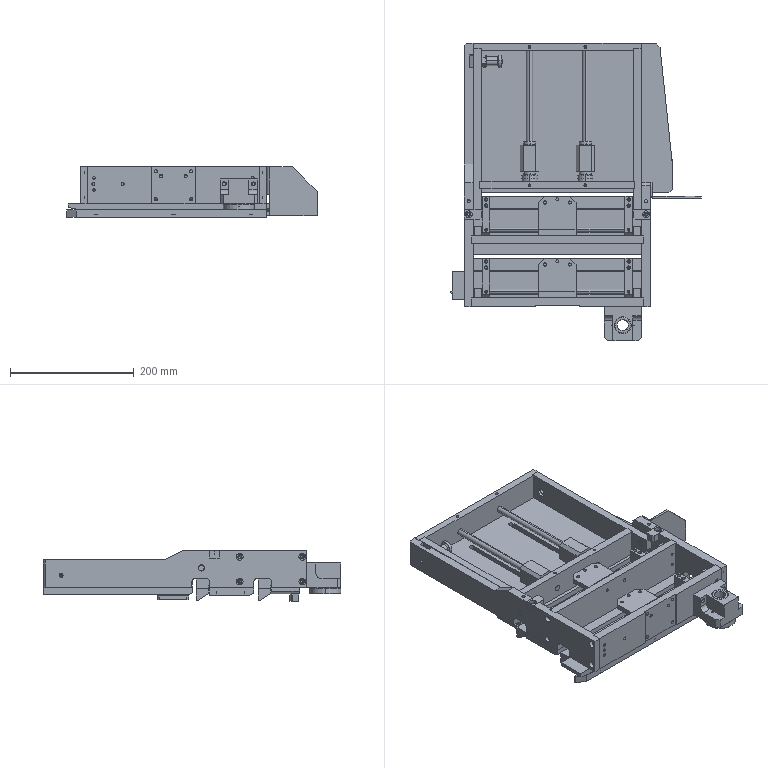Assembly | SolidWorks | mm | 48 component files | 48 solids | 1236 faces | box 404 x 480 x 82 mm | volume 3316165 mm3 | cylinder 579 | plane 451 | cone 200 | torus 4 | sphere 2 | commonest cylinder face diameters 5 x80 4.2 x78 10 x76 5.5 x62 6.6 x44 11 x42 12 x38 8 x28
Bill of materials:
LML10UU | 2 |  | Hollow cylindrical tube/sleeve with a through bore, chamfered ends and two shallow circumferential grooves near each end.
OPW-05-001 | 1 |  | Thick flat plate with an irregular stepped outline: a rectangular notch in one long edge, rounded-corner cutouts in the opposite edge, a chamfered corner, and several through holes including one larger hole near one end.
OPW-05-002 | 1 |  | Long thick bar/plate with a stepped and sloped top profile, rectangular notch, two rounded cutouts on the lower edge, multiple small through holes, one larger hole, and a rectangular pocket/recess near one end.
OPW-05-003 | 1 |  | Long rectangular bar with a shallow step/recess on one face in the middle section and a pattern of small holes on the main face plus two larger holes on each end face.
OPW-05-005 | 1 |  | Plain long rectangular bar with six small holes on the main face and two blind holes in each end face.
OPW-05-006 | 1 |  | Thin flat rectangular plate with one angled/chamfered corner, six small through holes and two larger holes that appear counterbored or larger near the ends.
OPW-05-007 | 1 |  | Thin flat plate of roughly rectangular outline with one long tapered/angled edge and chamfered corners, two long parallel slots, and six small holes along two opposite edges.
OPW-05-008 | 1 |  | Thin flat rectangular frame-like plate with three rounded-rectangular through windows separated by narrow webs, each web having two small holes, and chamfered outer corners.
OPW-05-010 | 1 |  | Prismatic block with a large vertical through bore, a raised central section with a curved (radiused) inner transition, stepped side ledges, horizontal cross holes, and chamfered corners on one end.
OPW-05-011 | 1 | Brass | Flanged cylindrical bushing: a hollow cylindrical body with a coaxial bore and a round flange at one end with four equally spaced through holes.
OPW-05-014 | 1 |  | Long slender rectangular bar with one angled/pointed end and three evenly spaced small holes along its length.
OPW-05-033 | 1 |  | Bent sheet-metal bracket with an L-shaped cross-section: a larger plate with an angled corner and a short perpendicular flange containing two holes.
STB-08-024 | 1 |  | Axisymmetric part with a hexagonal body at one end and a stepped cylindrical shank; a bore runs through along the axis.
STB-08-025 | 1 |  | Long cylindrical pin with a single raised annular collar near one end.
STB-08-026 | 1 |  | Short hollow cylindrical ring or sleeve with a central through bore.
STB-08-027 | 1 |  | Headed pin: a plain cylindrical shank with a larger-diameter head that has a domed outer face.
STB-08-005 | 1 |  | Long, thin, flat rectangular bar with a group of holes at each end and small holes along its length.
STB-08-007 | 2 | Brass | Long, slender prismatic bar with a non-rectangular cross-section (one sloped side ending in a rounded tip) and several holes.
STB-08-008 | 4 |  | Rectangular block with two parallel holes in one face and one larger perpendicular hole in an adjacent face.
STB-08-009 | 4 |  | Elongated rectangular block with one end chamfered, a transverse through hole at that end, top holes, and a stepped underside.
STB-08-010 | 2 |  | Long, slender, plain cylindrical rod.
STB-08-011 | 2 |  | Block with an L-shaped side profile: a thicker upright section at one end and a thinner base, with chamfered plan corners and several holes.
STB-08-015 | 2 |  | Solid plain cylinder with chamfered edges at both ends.
STB-08-020 | 2 |  | Long, slender, plain cylindrical rod, similar in form to a thin pin or wire segment.
STB-08-021 | 2 |  | Prismatic block with a large cylindrical through-bore along its length; the cross-section is a rectangle with two chamfered top corners, and a narrower rectangular tab hangs below it. The tab runs only part of the block's length, so the side profile is L-shaped.
STB-08-022 | 4 |  | Flat annular ring (washer-like disc) with a concentric central through-hole and plain cylindrical outer and inner surfaces.
STB-08-042 | 1 | 6061 Alloy | Long, thin rectangular bar. One end has a stepped L-shaped notch with a small chamfer and an inside fillet. There is one larger through-hole near each end and two smaller through-holes next to the notched end. A small raised or stepped tab detail sits near the notched end on one side face.
STB-08-042JX | 1 | 6061 Alloy | Long, thin rectangular bar with an L-shaped notch at one end (small chamfer and inside fillet). It has a larger through-hole near each end and two smaller through-holes beside the notched end. A small step appears on the face opposite the one seen on the similar part.
STB-08-043 | 1 | 6061 Alloy | Long rectangular bar with two through-holes in the main face, spaced along its length. It also has two small holes in the top narrow edge and two small holes in one end face.
STB-08-044 | 1 |  | Long rectangular bar with stepped (rebated) ends: a narrower raised strip runs along one long face between the end steps. It has two through-holes in the main face, two small holes near each end of the face, two small holes in the top edge, and small holes in both end faces.
STB-08-045 | 2 |  | Rectangular block with two chamfered corners at one end in plan view and a counterbored vertical through-hole near the other end.
Mates:
1. concentric | OPW-05-003-1 face at (-243.904, 48.999, -20) dir (-1, 0, 0) r 2.5 | OPW-05-002-1 face at (-254.904, 48.999, -20) dir (-1, 0, 0) r 3.3
2. concentric | OPW-05-003-1 face at (-243.904, 48.999, 20) dir (-1, 0, 0) r 2.5 | OPW-05-002-1 face at (-254.904, 48.999, 20) dir (-1, 0, 0) r 3.3
3. coincident | OPW-05-003-1 face at (-243.904, 55.999, -30) dir (-1, 0, 0) | OPW-05-002-1 face at (-243.904, 55.999, -30) dir (1, 0, 0)
4. concentric | OPW-05-003-1 face at (34.096, 48.999, -20) dir (1, 0, 0) r 2.5 | OPW-05-001-1 face at (45.096, 48.999, -20) dir (1, 0, 0) r 5.5
5. concentric | OPW-05-003-1 face at (34.096, 48.999, 20) dir (1, 0, 0) r 2.5 | OPW-05-001-1 face at (45.096, 48.999, 20) dir (1, 0, 0) r 5.5
6. coincident | OPW-05-003-1 face at (34.096, 55.999, -30) dir (1, 0, 0) | OPW-05-001-1 face at (34.096, 55.999, -30) dir (-1, 0, 0)
7. concentric | OPW-05-002-1 face at (-254.904, 149.999, 20) dir (-1, 0, 0) r 5.5 | OPW-05-005-1 face at (-243.904, 149.999, 20) dir (-1, 0, 0) r 2.5
8. concentric | OPW-05-002-1 face at (-254.904, 149.999, -20) dir (-1, 0, 0) r 5.5 | OPW-05-005-1 face at (-243.904, 149.999, -20) dir (-1, 0, 0) r 2.5
9. coincident | OPW-05-002-1 face at (-243.904, 143.999, 30) dir (1, 0, 0) | OPW-05-005-1 face at (-243.904, 155.999, -30) dir (-1, 0, 0)
10. concentric | OPW-05-003-1 face at (-232.904, 55.999, -8) dir (0, 1, 0) r 2.1 | STB-08-008-1 face at (-232.904, 71.999, -8) dir (0, 1, 0) r 2.75
11. concentric | OPW-05-003-1 face at (-232.904, 55.999, 12) dir (0, 1, 0) r 2.1 | STB-08-008-1 face at (-232.904, 71.999, 12) dir (0, 1, 0) r 2.75
12. coincident | OPW-05-003-1 face at (-243.904, 55.999, 30) dir (0, 1, 0) | STB-08-008-1 face at (-238.904, 55.999, -27) dir (0, -1, 0)
13. concentric | OPW-05-003-1 face at (23.096, 55.999, 12) dir (0, 1, 0) r 2.1 | STB-08-008-2 face at (23.096, 71.999, 12) dir (0, 1, 0) r 2.75
14. concentric | OPW-05-003-1 face at (23.096, 55.999, -8) dir (0, 1, 0) r 2.1 | STB-08-008-2 face at (23.096, 71.999, -8) dir (0, 1, 0) r 2.75
15. coincident | OPW-05-003-1 face at (-243.904, 55.999, 30) dir (0, 1, 0) | STB-08-008-2 face at (17.096, 55.999, -27) dir (0, -1, 0)
16. concentric | OPW-05-005-1 face at (23.096, 155.999, 12) dir (0, 1, 0) r 2.1 | STB-08-008-4 face at (23.096, 171.999, 12) dir (0, 1, 0) r 2.75
17. concentric | OPW-05-005-1 face at (23.096, 155.999, -8) dir (0, 1, 0) r 2.1 | STB-08-008-4 face at (23.096, 171.999, -8) dir (0, 1, 0) r 2.75
18. coincident | OPW-05-005-1 face at (-243.904, 155.999, 30) dir (0, 1, 0) | STB-08-008-4 face at (17.096, 155.999, -27) dir (0, -1, 0)
19. concentric | OPW-05-005-1 face at (-232.904, 155.999, -8) dir (0, 1, 0) r 2.1 | STB-08-008-3 face at (-232.904, 171.999, -8) dir (0, 1, 0) r 2.75
20. concentric | OPW-05-005-1 face at (-232.904, 155.999, 12) dir (0, 1, 0) r 2.1 | STB-08-008-3 face at (-232.904, 171.999, 12) dir (0, 1, 0) r 2.75
21. coincident | OPW-05-005-1 face at (-243.904, 155.999, 30) dir (0, 1, 0) | STB-08-008-3 face at (-238.904, 155.999, -27) dir (0, -1, 0)
22. concentric | STB-08-010-1 face at (29.096, 65.999, -19) dir (-1, 0, 0) r 4 | STB-08-008-2 face at (17.095, 65.999, -19) dir (1, 0, 0) r 4
23. coincident | STB-08-010-1 face at (29.096, 65.999, -19) dir (1, 0, 0) | STB-08-008-2 face at (29.096, 55.999, -27) dir (1, 0, 0)
24. concentric | STB-08-009-1 face at (-225.905, 65.999, -19) dir (1, 0, 0) r 4 | STB-08-010-1 face at (29.096, 65.999, -19) dir (-1, 0, 0) r 4
25. concentric | STB-08-007-1 face at (-219.904, 114.999, -31) dir (0, 0, 1) r 2.1 | STB-08-009-1 face at (-219.904, 114.999, -9) dir (0, 0, 1) r 2.75
26. concentric | STB-08-007-1 face at (-219.904, 104.999, -31) dir (0, 0, 1) r 2.1 | STB-08-009-1 face at (-219.904, 104.999, -9) dir (0, 0, 1) r 2.75
27. coincident | STB-08-007-1 face at (-254.904, 119.999, -31) dir (0, 0, 1) | STB-08-009-1 face at (-225.904, 57.999, -31) dir (0, 0, -1)
28. concentric | STB-08-007-1 face at (10.096, 104.999, -31) dir (0, 0, 1) r 2.1 | STB-08-009-2 face at (10.096, 104.999, -9) dir (0, 0, 1) r 2.75
29. concentric | STB-08-007-1 face at (10.096, 114.999, -31) dir (0, 0, 1) r 2.1 | STB-08-009-2 face at (10.096, 114.999, -9) dir (0, 0, 1) r 2.75
30. coincident | STB-08-007-1 face at (-254.904, 119.999, -31) dir (0, 0, 1) | STB-08-009-2 edge at (10.096, 104.999, -31) dir (0, 0, 1) r 2.75
31. distance | STB-08-008-1 face at (-226.904, 55.999, -27) dir (1, 0, 0) | STB-08-009-1 face at (-225.904, 119.999, -9) dir (-1, 0, 0)
32. parallel | OPW-05-002-1 face at (-240.903, 98.999, -30) dir (0, 1, 0) | STB-08-007-1 face at (-254.904, 119.999, -51) dir (0, 1, 0)
33. concentric | OPW-05-003-1 face at (-124.904, 55.999, 15) dir (0, 1, 0) r 2.5 | STB-08-011-1 face at (-124.904, 65.999, 15) dir (0, 1, 0) r 3.5
34. concentric | OPW-05-003-1 face at (-84.904, 55.999, 15) dir (0, 1, 0) r 2.5 | STB-08-011-1 face at (-84.904, 65.999, 15) dir (0, 1, 0) r 3.5
35. coincident | OPW-05-003-1 face at (-243.904, 55.999, 30) dir (0, 1, 0) | STB-08-011-1 face at (-134.904, 55.999, 1) dir (0, -1, 0)
36. concentric | STB-08-008-3 face at (-238.905, 165.999, -19) dir (1, 0, 0) r 4 | STB-08-010-2 face at (29.096, 165.999, -19) dir (-1, 0, 0) r 4
37. coincident | STB-08-008-3 face at (-238.904, 155.999, -27) dir (-1, 0, 0) | STB-08-010-2 face at (-238.904, 165.999, -19) dir (-1, 0, 0)
38. concentric | STB-08-009-3 face at (-225.905, 165.999, -19) dir (1, 0, 0) r 4 | STB-08-010-2 face at (29.096, 165.999, -19) dir (-1, 0, 0) r 4
39. concentric | STB-08-007-2 face at (-219.904, 214.999, -31) dir (0, 0, 1) r 2.1 | STB-08-009-3 face at (-219.904, 214.999, -9) dir (0, 0, 1) r 2.75
40. concentric | STB-08-007-2 face at (10.096, 214.999, -31) dir (0, 0, 1) r 2.1 | STB-08-009-4 face at (10.096, 214.999, -9) dir (0, 0, 1) r 2.75
41. coincident | STB-08-009-4 edge at (4.096, 165.999, -19) dir (-1, 0, 0) r 4 | STB-08-010-2 face at (29.096, 165.999, -19) dir (-1, 0, 0) r 4
42. coincident | STB-08-007-2 face at (-254.904, 219.999, -31) dir (0, 0, 1) | STB-08-009-4 edge at (10.096, 204.999, -31) dir (0, 0, 1) r 2.75
43. parallel | OPW-05-002-1 face at (-240.903, 198.999, -30) dir (0, 1, 0) | STB-08-007-2 face at (-254.904, 219.999, -51) dir (0, 1, 0)
44. coincident | STB-08-007-1 face at (-254.904, 99.999, -51) dir (-1, 0, 0) | STB-08-007-2 face at (-254.904, 199.999, -51) dir (-1, 0, 0)
45. concentric | OPW-05-005-1 face at (-84.904, 155.999, 15) dir (0, 1, 0) r 2.5 | STB-08-011-2 face at (-84.904, 165.999, 15) dir (0, 1, 0) r 3.5
46. concentric | OPW-05-005-1 face at (-124.904, 155.999, 15) dir (0, 1, 0) r 2.5 | STB-08-011-2 face at (-124.904, 165.999, 15) dir (0, 1, 0) r 3.5
47. coincident | OPW-05-005-1 face at (-243.904, 155.999, 30) dir (0, 1, 0) | STB-08-011-2 face at (-134.904, 155.999, 1) dir (0, -1, 0)
48. concentric | OPW-05-001-1 face at (38.096, 90.999, -30) dir (0, 0, -1) r 2.5 | STB-08-005-1 face at (38.096, 90.999, -40) dir (0, 0, -1) r 5.5
49. concentric | OPW-05-001-1 face at (38.096, 72.999, -30) dir (0, 0, -1) r 2.5 | STB-08-005-1 face at (38.096, 72.999, -40) dir (0, 0, -1) r 5.5
50. coincident | OPW-05-001-1 face at (31.096, 241.999, -30) dir (0, 0, -1) | STB-08-005-1 face at (45.096, 53.999, -30) dir (0, 0, 1)
51. concentric | STB-08-005-1 face at (20.096, 60.999, -40) dir (0, 0, -1) r 2.1 | OPW-05-014-1 face at (20.096, 60.999, -52) dir (0, 0, -1) r 2.75
52. concentric | STB-08-005-1 face at (-104.904, 60.999, -40) dir (0, 0, -1) r 2.1 | OPW-05-014-1 face at (-104.904, 60.999, -52) dir (0, 0, -1) r 2.75
53. coincident | STB-08-005-1 face at (45.096, 53.999, -40) dir (0, 0, -1) | OPW-05-014-1 face at (45.096, 54.999, -40) dir (0, 0, 1)
54. concentric | OPW-05-002-1 face at (-247.904, 190.999, 18) dir (0, 0, 1) r 2.5 | STB-08-045-1 face at (-247.904, 190.999, 30) dir (0, 0, 1) r 3.3
55. coincident | OPW-05-002-1 face at (-254.904, 198.999, 18) dir (0, 0, 1) | STB-08-045-1 face at (-254.904, 182.999, 18) dir (0, 0, -1)
56. coincident | OPW-05-002-1 face at (-254.904, 41.999, -30) dir (-1, 0, 0) | STB-08-045-1 face at (-254.904, 198.999, 30) dir (-1, 0, 0)
57. concentric | OPW-05-001-1 face at (38.096, 190.999, 18) dir (0, 0, 1) r 2.5 | STB-08-045-2 face at (38.096, 190.999, 30) dir (0, 0, 1) r 3.3
58. coincident | OPW-05-001-1 face at (31.095, 198.999, 18) dir (0, 0, 1) | STB-08-045-2 face at (45.096, 198.999, 18) dir (0, 0, -1)
59. coincident | OPW-05-001-1 face at (45.096, 41.999, -30) dir (1, 0, 0) | STB-08-045-2 face at (45.096, 182.999, 30) dir (1, 0, 0)
60. concentric | OPW-05-002-1 face at (-247.904, 186.999, -30) dir (0, 0, -1) r 2.5 | OPW-05-006-1 face at (-247.904, 186.999, -42) dir (0, 0, -1) r 3.3
61. concentric | OPW-05-002-1 face at (-247.904, 141.999, -30) dir (0, 0, -1) r 2.5 | OPW-05-006-1 face at (-247.904, 141.999, -42) dir (0, 0, -1) r 3.3
62. coincident | OPW-05-002-1 face at (-254.904, 466.999, -30) dir (0, 0, -1) | OPW-05-006-1 face at (45.096, 126.999, -30) dir (0, 0, 1)
63. concentric | OPW-05-002-1 face at (-254.905, 211.999, 2) dir (1, 0, 0) r 5 | STB-08-042-1 face at (-227.903, 211.999, 2) dir (-1, 0, 0) r 6
64. concentric | OPW-05-001-1 face at (31.095, 211.999, 2) dir (1, 0, 0) r 5 | STB-08-042JX-1 face at (18.095, 211.999, 2) dir (1, 0, 0) r 6
65. concentric | STB-08-042-1 face at (-233.904, 457.999, 5.5) dir (0, 1, 0) r 2.1 | STB-08-044-1 face at (-233.904, 466.999, 5.5) dir (0, 1, 0) r 5
66. concentric | STB-08-042-1 face at (-233.904, 457.999, -19.5) dir (0, 1, 0) r 2.1 | STB-08-044-1 face at (-233.904, 466.999, -19.5) dir (0, 1, 0) r 2.75
67. coincident | STB-08-042-1 face at (-239.904, 457.999, -29) dir (0, 1, 0) | STB-08-044-1 face at (-239.904, 457.999, -29.001) dir (0, -1, 0)
68. concentric | STB-08-042JX-1 face at (24.096, 457.999, -19.5) dir (0, 1, 0) r 2.1 | STB-08-044-1 face at (24.096, 466.999, -19.5) dir (0, 1, 0) r 5
69. concentric | STB-08-042JX-1 face at (24.096, 457.999, 5.5) dir (0, 1, 0) r 2.1 | STB-08-044-1 face at (24.096, 466.999, 5.5) dir (0, 1, 0) r 2.75
70. distance | STB-08-042-1 face at (-239.904, 197.999, -29) dir (-1, 0, 0) | OPW-05-002-1 face at (-240.904, 41.999, -30) dir (1, 0, 0)
71. concentric | STB-08-042-1 face at (-239.904, 237.999, 5.5) dir (-1, 0, 0) r 2.75 | STB-08-043-1 face at (-229.904, 237.999, 5.5) dir (-1, 0, 0) r 2.1
72. concentric | STB-08-042-1 face at (-239.904, 237.999, -19.5) dir (-1, 0, 0) r 2.75 | STB-08-043-1 face at (-229.904, 237.999, -19.5) dir (-1, 0, 0) r 2.1
73. coincident | STB-08-042-1 face at (-229.904, 231.999, 15) dir (1, 0, 0) | STB-08-043-1 face at (-229.904, 243.999, -29) dir (-1, 0, 0)
74. concentric | OPW-05-002-1 face at (-254.905, 437.999, -10) dir (1, 0, 0) r 3 | STB-08-042-1 face at (-231.904, 437.999, -10) dir (1, 0, 0) r 6
75. concentric | STB-08-044-1 face at (-149.904, 454.998, -12) dir (0, 1, 0) r 5 | STB-08-020-1 face at (-149.904, 466.999, -12) dir (0, -1, 0) r 5
76. coincident | STB-08-044-1 face at (-239.904, 466.999, -29) dir (0, 1, 0) | STB-08-020-1 face at (-149.904, 466.999, -12) dir (0, 1, 0)
77. concentric | STB-08-044-1 face at (-59.904, 454.998, -12) dir (0, 1, 0) r 5 | STB-08-020-2 face at (-59.904, 466.999, -12) dir (0, -1, 0) r 5
78. coincident | STB-08-044-1 face at (-239.904, 466.999, -29) dir (0, 1, 0) | STB-08-020-2 face at (-59.904, 466.999, -12) dir (0, 1, 0)
79. concentric | STB-08-020-1 face at (-149.904, 466.999, -12) dir (0, -1, 0) r 5 | STB-08-022-1 face at (-149.904, 243.998, -12) dir (0, 1, 0) r 5
80. coincident | STB-08-043-1 face at (-229.904, 243.999, -29) dir (0, 1, 0) | STB-08-022-1 face at (-149.904, 243.999, -12) dir (0, -1, 0)
81. concentric | STB-08-020-2 face at (-59.904, 466.999, -12) dir (0, -1, 0) r 5 | STB-08-022-2 face at (-59.904, 243.998, -12) dir (0, 1, 0) r 5
82. coincident | STB-08-043-1 face at (-229.904, 243.999, -29) dir (0, 1, 0) | STB-08-022-2 face at (-59.904, 243.999, -12) dir (0, -1, 0)
83. concentric | STB-08-020-1 face at (-149.904, 466.999, -12) dir (0, -1, 0) r 5 | STB-08-022-3 face at (-149.904, 253.999, -12) dir (0, -1, 0) r 12.5
84. coincident | STB-08-022-1 face at (-149.904, 248.999, -12) dir (0, 1, 0) | STB-08-022-3 face at (-149.904, 248.999, -12) dir (0, -1, 0)
85. concentric | STB-08-020-2 face at (-59.904, 466.999, -12) dir (0, -1, 0) r 5 | STB-08-022-4 face at (-59.904, 253.999, -12) dir (0, -1, 0) r 12.5
86. coincident | STB-08-022-2 face at (-59.904, 248.999, -12) dir (0, 1, 0) | STB-08-022-4 face at (-59.904, 248.999, -12) dir (0, -1, 0)
87. concentric | STB-08-020-1 face at (-149.904, 466.999, -12) dir (0, -1, 0) r 5 | STB-08-021-1 face at (-149.904, 260.498, -12) dir (0, 1, 0) r 9.5
88. concentric | STB-08-020-2 face at (-59.904, 466.999, -12) dir (0, -1, 0) r 5 | STB-08-021-2 face at (-59.904, 260.498, -12) dir (0, 1, 0) r 9.5
89. concentric | STB-08-020-1 face at (-149.904, 466.999, -12) dir (0, -1, 0) r 5 | LML10UU-1 face at (-149.904, 308.999, -12) dir (0, -1, 0) r 9.5
90. coincident | STB-08-021-1 face at (-164.904, 260.499, 3) dir (0, -1, 0) | LML10UU-1 face at (-140.617, 260.499, -14.002) dir (0, -1, 0)
91. coincident | STB-08-022-3 face at (-149.904, 253.999, -12) dir (0, 1, 0) | LML10UU-1 face at (-149.904, 253.999, -12) dir (0, -1, 0)
92. concentric | STB-08-020-2 face at (-59.904, 466.999, -12) dir (0, -1, 0) r 5 | LML10UU-2 face at (-59.904, 308.999, -12) dir (0, -1, 0) r 9.5
93. coincident | STB-08-021-2 face at (-74.904, 260.499, 3) dir (0, -1, 0) | LML10UU-2 face at (-50.617, 260.499, -14.002) dir (0, -1, 0)
94. coincident | STB-08-022-4 face at (-59.904, 253.999, -12) dir (0, 1, 0) | LML10UU-2 face at (-59.904, 253.999, -12) dir (0, -1, 0)
95. concentric | STB-08-042-1 face at (-231.904, 437.999, -10) dir (1, 0, 0) r 6 | STB-08-000-3-1/STB-08-024-1 face at (-227.904, 437.999, -10) dir (-1, 0, 0) r 7
96. coincident | STB-08-042-1 face at (-227.904, 197.999, -29) dir (1, 0, 0) | STB-08-000-3-1/STB-08-024-1 face at (-227.904, 437.999, -10) dir (-1, 0, 0)
97. concentric | OPW-05-002-1 face at (-254.905, 211.999, 2) dir (1, 0, 0) r 5 | STB-08-015-1 face at (-227.904, 211.999, 2) dir (-1, 0, 0) r 5
98. coincident | OPW-05-002-1 face at (-254.904, 41.999, -30) dir (-1, 0, 0) | STB-08-015-1 face at (-254.904, 211.999, 2) dir (-1, 0, 0)
99. coincident | STB-08-044-1 face at (30.096, 466.999, -29) dir (0, 0, -1) | OPW-05-007-1 face at (-239.904, 225.999, -29) dir (0, 0, 1)
100. concentric | STB-08-043-1 face at (-194.904, 237.999, -29) dir (0, 0, -1) r 1.65 | OPW-05-007-1 face at (-194.904, 237.999, -41) dir (0, 0, -1) r 2.25
101. concentric | STB-08-043-1 face at (-104.904, 237.999, -29) dir (0, 0, -1) r 1.65 | OPW-05-007-1 face at (-104.904, 237.999, -41) dir (0, 0, -1) r 2.25
102. concentric | STB-08-021-1 face at (-149.904, 276.499, -45) dir (0, 0, -1) r 1.65 | OPW-05-008-1 face at (-149.904, 276.499, -49) dir (0, 0, 1) r 785.398
103. concentric | STB-08-021-1 face at (-149.904, 266.499, -45) dir (0, 0, -1) r 1.65 | OPW-05-008-1 face at (-149.904, 266.499, -49) dir (0, 0, 1) r 785.398
104. coincident | STB-08-021-1 face at (-164.904, 302.499, -45) dir (0, 0, -1) | OPW-05-008-1 face at (-153.404, 232.499, -45) dir (0, 0, 1)
105. concentric | STB-08-021-2 face at (-59.904, 276.499, -45) dir (0, 0, -1) r 1.65 | OPW-05-008-1 face at (-59.904, 276.499, -49) dir (0, 0, -1) r 2.25
106. concentric | OPW-05-001-1 face at (31.095, 211.999, 2) dir (1, 0, 0) r 5 | STB-08-015-2 face at (45.096, 211.999, 2) dir (-1, 0, 0) r 5
107. coincident | OPW-05-001-1 face at (45.096, 41.999, -30) dir (1, 0, 0) | STB-08-015-2 face at (45.096, 211.999, 2) dir (1, 0, 0)
108. concentric | OPW-05-003-1 face at (24.096, 41.999, 2) dir (0, -1, 0) r 2.5 | OPW-05-010-1 face at (24.096, 26.999, 2) dir (0, -1, 0) r 3.3
109. concentric | OPW-05-003-1 face at (-22.904, 41.999, 2) dir (0, -1, 0) r 2.5 | OPW-05-010-1 face at (-22.904, 26.999, 2) dir (0, -1, 0) r 3.3
110. coincident | OPW-05-003-1 face at (-243.904, 41.999, 30) dir (0, -1, 0) | OPW-05-010-1 face at (30.596, 41.999, -30) dir (0, 1, 0)
111. concentric | OPW-05-010-1 face at (0.5965, 11.999, 10.001) dir (0, 0, -1) r 13.5 | OPW-05-011-1 face at (0.5965, 11.999, -40) dir (0, 0, -1) r 8.75
112. concentric | OPW-05-010-1 face at (0.5965, 29.999, -30) dir (0, 0, -1) r 2.1 | OPW-05-011-1 face at (0.5965, 29.999, -40) dir (0, 0, -1) r 5
113. coincident | OPW-05-010-1 face at (30.596, -13.001, -30) dir (0, 0, -1) | OPW-05-011-1 face at (0.5965, 11.999, -30) dir (0, 0, 1)
114. concentric | OPW-05-001-1 face at (45.096, 229.499, -5) dir (1, 0, 0) r 2.5 | OPW-05-033-1 face at (48.096, 229.499, -5) dir (1, 0, 0) r 3.25
115. concentric | OPW-05-001-1 face at (45.096, 229.499, 20) dir (1, 0, 0) r 2.5 | OPW-05-033-1 face at (48.096, 229.499, 20) dir (1, 0, 0) r 3.25
116. coincident | OPW-05-001-1 face at (45.096, 41.999, -30) dir (1, 0, 0) | OPW-05-033-1 face at (45.096, 241.999, 30) dir (-1, 0, 0)
117. concentric | STB-08-024-1 face at (-109.421, 15.093, 0) dir (-1, 0, 0) r 3 | STB-08-025-1 face at (-126.422, 15.093, 0) dir (-1, 0, 0) r 3
118. coincident | STB-08-024-1 face at (-126.422, 15.093, 0) dir (1, 0, 0) | STB-08-025-1 face at (-126.422, 15.093, 0) dir (-1, 0, 0)
119. concentric | STB-08-024-1 face at (-113.422, 15.093, 0) dir (1, 0, 0) r 5 | STB-08-026-2 face at (-109.422, 15.093, 0) dir (-1, 0, 0) r 5
120. coincident | STB-08-024-1 face at (-113.422, 15.093, 0) dir (1, 0, 0) | STB-08-026-2 face at (-113.422, 15.093, 0) dir (-1, 0, 0)
121. concentric | STB-08-025-1 face at (-124.422, 15.093, 0) dir (1, 0, 0) r 3 | STB-08-027-1 face at (-109.422, 15.093, 0) dir (-1, 0, 0) r 3
122. coincident | STB-08-024-1 face at (-109.422, 24.907, 0) dir (1, 0, 0) | STB-08-027-1 face at (-109.422, 15.093, 0) dir (-1, 0, 0)